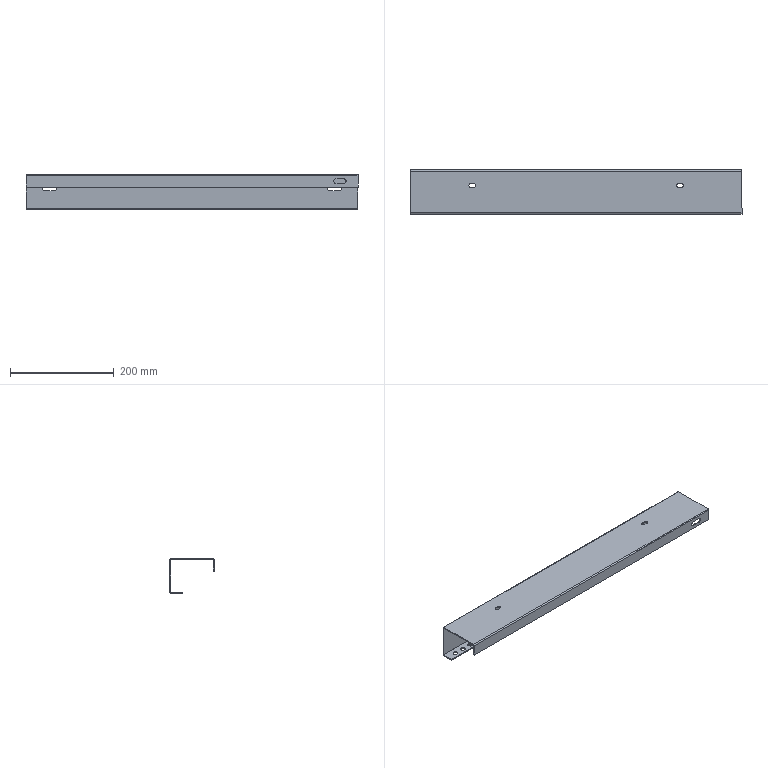Component | SolidWorks | KSHE-016.005-1 | 1 solid | 114 faces | volume 240533 mm3 | cylinder 80 | plane 34 | commonest cylinder face diameters 9 x64 7 x6 13 x4 4.2 x3 0.2 x3